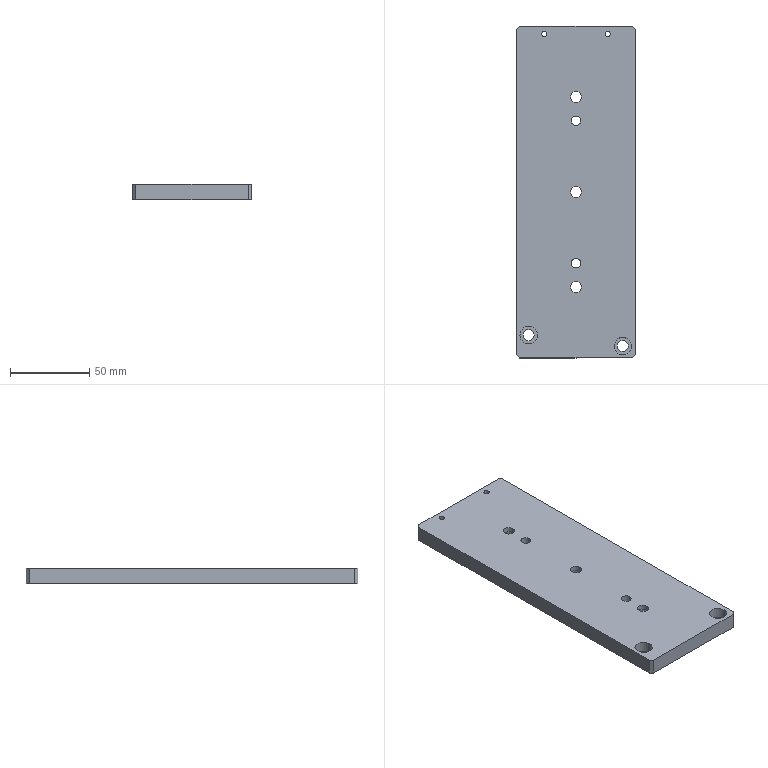Component | SolidWorks | 8TC-A17001-90-05EdgePressingBasePlate-1 | 1 solid | 115 faces | box 75 x 210 x 10 mm | volume 151671 mm3 | cylinder 64 | cone 36 | plane 15 | commonest cylinder face diameters 2.5 x28 6 x12 11 x10 7 x10 3.3 x4 | material A3
build123d program:
from build123d import *

# Parameters (mm, degrees)
SKETCH1_W                                          = 75
SKETCH1_H                                          = 210
BOSS_EXTRUDE1_DEPTH                                = 10
HOLE_SIZE_ACCORDING_TO_TYPE_1_HEX_SOCK_D           = 7
HOLE_SIZE_ACCORDING_TO_TYPE_1_HEX_SOCK_DEPTH       = 18
HOLE_SIZE_ACCORDING_TO_TYPE_1_HEX_SOCK_CBORE_D     = 11
HOLE_SIZE_ACCORDING_TO_TYPE_1_HEX_SOCK_CBORE_DEPTH = 6.8
HOLE_SIZE_ACCORDING_TO_TYPE_1_HEX_SOCK_TIP         = 2.103
M3_TAPPED_HOLE1_D                                  = 2.5
M3_TAPPED_HOLE1_DEPTH                              = 7.5
M3_TAPPED_HOLE1_TIP                                = 0.7511
M4_TAPPED_HOLE1_D                                  = 3.3
M4_TAPPED_HOLE1_DEPTH                              = 10.1
M4_TAPPED_HOLE1_TIP                                = 0.9914
HOLE_SIZE_ACCORDING_TO_HEXAGON_SOCKET_D            = 7
HOLE_SIZE_ACCORDING_TO_HEXAGON_SOCKET_DEPTH        = 10.1
HOLE_SIZE_ACCORDING_TO_HEXAGON_SOCKET_CBORE_D      = 11
HOLE_SIZE_ACCORDING_TO_HEXAGON_SOCKET_CBORE_DEPTH  = 6.8
HOLE_SIZE_ACCORDING_TO_HEXAGON_SOCKET_TIP          = 2.103
CHAMFER1_SIZE                                      = 2
SIZE_MM_DOWEL_PIN_HOLE_1_D                         = 6
SIZE_MM_DOWEL_PIN_HOLE_1_DEPTH                     = 10
SIZE_MM_DOWEL_PIN_HOLE_1_TIP                       = 1.803
SIZE_MM_DOWEL_PIN_HOLE2_D                          = 6
SIZE_MM_DOWEL_PIN_HOLE2_DEPTH                      = 5
SIZE_MM_DOWEL_PIN_HOLE2_TIP                        = 1.803


with BuildPart() as part:
    # Sketch1 → Boss-Extrude1 (new body)
    with BuildSketch(Plane.XY):
        Rectangle(SKETCH1_W, SKETCH1_H)
    extrude(amount=BOSS_EXTRUDE1_DEPTH)

    # Hole Size _according to_ Type 1 Hex Sock
    with Locations(Plane(origin=(0, 0, 0), x_dir=(-1, 0, 0), z_dir=(0, 0, -1))):
        with Locations((0, 0), (0, 60), (0, -60)):
            CounterBoreHole(HOLE_SIZE_ACCORDING_TO_TYPE_1_HEX_SOCK_D / 2, HOLE_SIZE_ACCORDING_TO_TYPE_1_HEX_SOCK_CBORE_D / 2, HOLE_SIZE_ACCORDING_TO_TYPE_1_HEX_SOCK_CBORE_DEPTH, depth=HOLE_SIZE_ACCORDING_TO_TYPE_1_HEX_SOCK_DEPTH)
            with Locations((0, 0, -(HOLE_SIZE_ACCORDING_TO_TYPE_1_HEX_SOCK_DEPTH + HOLE_SIZE_ACCORDING_TO_TYPE_1_HEX_SOCK_TIP / 2))):  # 118° drill point
                Cone(0, HOLE_SIZE_ACCORDING_TO_TYPE_1_HEX_SOCK_D / 2, HOLE_SIZE_ACCORDING_TO_TYPE_1_HEX_SOCK_TIP, mode=Mode.SUBTRACT)

    # M3 Tapped Hole1
    with Locations(Plane(origin=(0, 0, 0), x_dir=(-1, 0, 0), z_dir=(0, 0, -1))):
        with Locations((-24, -65), (-24, -40), (-24, -15), (-24, 10), (-24, 35), (-24, 60), (-24, 85), (24, -65), (24, -40), (24, -15), (24, 10), (24, 35), (24, 60), (24, 85)):
            Hole(M3_TAPPED_HOLE1_D / 2, depth=M3_TAPPED_HOLE1_DEPTH)
            with Locations((0, 0, -(M3_TAPPED_HOLE1_DEPTH + M3_TAPPED_HOLE1_TIP / 2))):  # 118° drill point
                Cone(0, M3_TAPPED_HOLE1_D / 2, M3_TAPPED_HOLE1_TIP, mode=Mode.SUBTRACT)

    # M4 Tapped Hole1
    with Locations(Plane(origin=(0, 0, 0), x_dir=(-1, 0, 0), z_dir=(0, 0, -1))):
        with Locations((20, 100), (-20, 100)):
            Hole(M4_TAPPED_HOLE1_D / 2, depth=M4_TAPPED_HOLE1_DEPTH)
            with Locations((0, 0, -(M4_TAPPED_HOLE1_DEPTH + M4_TAPPED_HOLE1_TIP / 2))):  # 118° drill point
                Cone(0, M4_TAPPED_HOLE1_D / 2, M4_TAPPED_HOLE1_TIP, mode=Mode.SUBTRACT)

    # Hole Size _ according to_ Hexagon Socket
    with Locations(Plane.XY.offset(10)):
        with Locations((-30, -90.5), (29.59, -97.5)):
            CounterBoreHole(HOLE_SIZE_ACCORDING_TO_HEXAGON_SOCKET_D / 2, HOLE_SIZE_ACCORDING_TO_HEXAGON_SOCKET_CBORE_D / 2, HOLE_SIZE_ACCORDING_TO_HEXAGON_SOCKET_CBORE_DEPTH, depth=HOLE_SIZE_ACCORDING_TO_HEXAGON_SOCKET_DEPTH)
            with Locations((0, 0, -(HOLE_SIZE_ACCORDING_TO_HEXAGON_SOCKET_DEPTH + HOLE_SIZE_ACCORDING_TO_HEXAGON_SOCKET_TIP / 2))):  # 118° drill point
                Cone(0, HOLE_SIZE_ACCORDING_TO_HEXAGON_SOCKET_D / 2, HOLE_SIZE_ACCORDING_TO_HEXAGON_SOCKET_TIP, mode=Mode.SUBTRACT)

    # Chamfer1
    chamfer1_edges = [part.edges().sort_by_distance(p)[0] for p in [
        (-37.5, 105, 5),
        (37.5, 105, 5),
        (37.5, -105, 5),
        (-37.5, -105, 5),
    ]]
    chamfer(chamfer1_edges, length=CHAMFER1_SIZE)

    # Size mm Dowel Pin Hole 1
    with Locations(Plane(origin=(0, 0, 0), x_dir=(-1, 0, 0), z_dir=(0, 0, -1))):
        with Locations((0, 45), (0, -45)):
            Hole(SIZE_MM_DOWEL_PIN_HOLE_1_D / 2, depth=SIZE_MM_DOWEL_PIN_HOLE_1_DEPTH)
            with Locations((0, 0, -(SIZE_MM_DOWEL_PIN_HOLE_1_DEPTH + SIZE_MM_DOWEL_PIN_HOLE_1_TIP / 2))):  # 118° drill point
                Cone(0, SIZE_MM_DOWEL_PIN_HOLE_1_D / 2, SIZE_MM_DOWEL_PIN_HOLE_1_TIP, mode=Mode.SUBTRACT)

    # Size mm Dowel Pin Hole2
    with Locations(Plane(origin=(0, 0, 0), x_dir=(-1, 0, 0), z_dir=(0, 0, -1))):
        with Locations((15, -65), (15, 85), (-15, 85), (-15, -65)):
            Hole(SIZE_MM_DOWEL_PIN_HOLE2_D / 2, depth=SIZE_MM_DOWEL_PIN_HOLE2_DEPTH)
            with Locations((0, 0, -(SIZE_MM_DOWEL_PIN_HOLE2_DEPTH + SIZE_MM_DOWEL_PIN_HOLE2_TIP / 2))):  # 118° drill point
                Cone(0, SIZE_MM_DOWEL_PIN_HOLE2_D / 2, SIZE_MM_DOWEL_PIN_HOLE2_TIP, mode=Mode.SUBTRACT)


solid = part.part